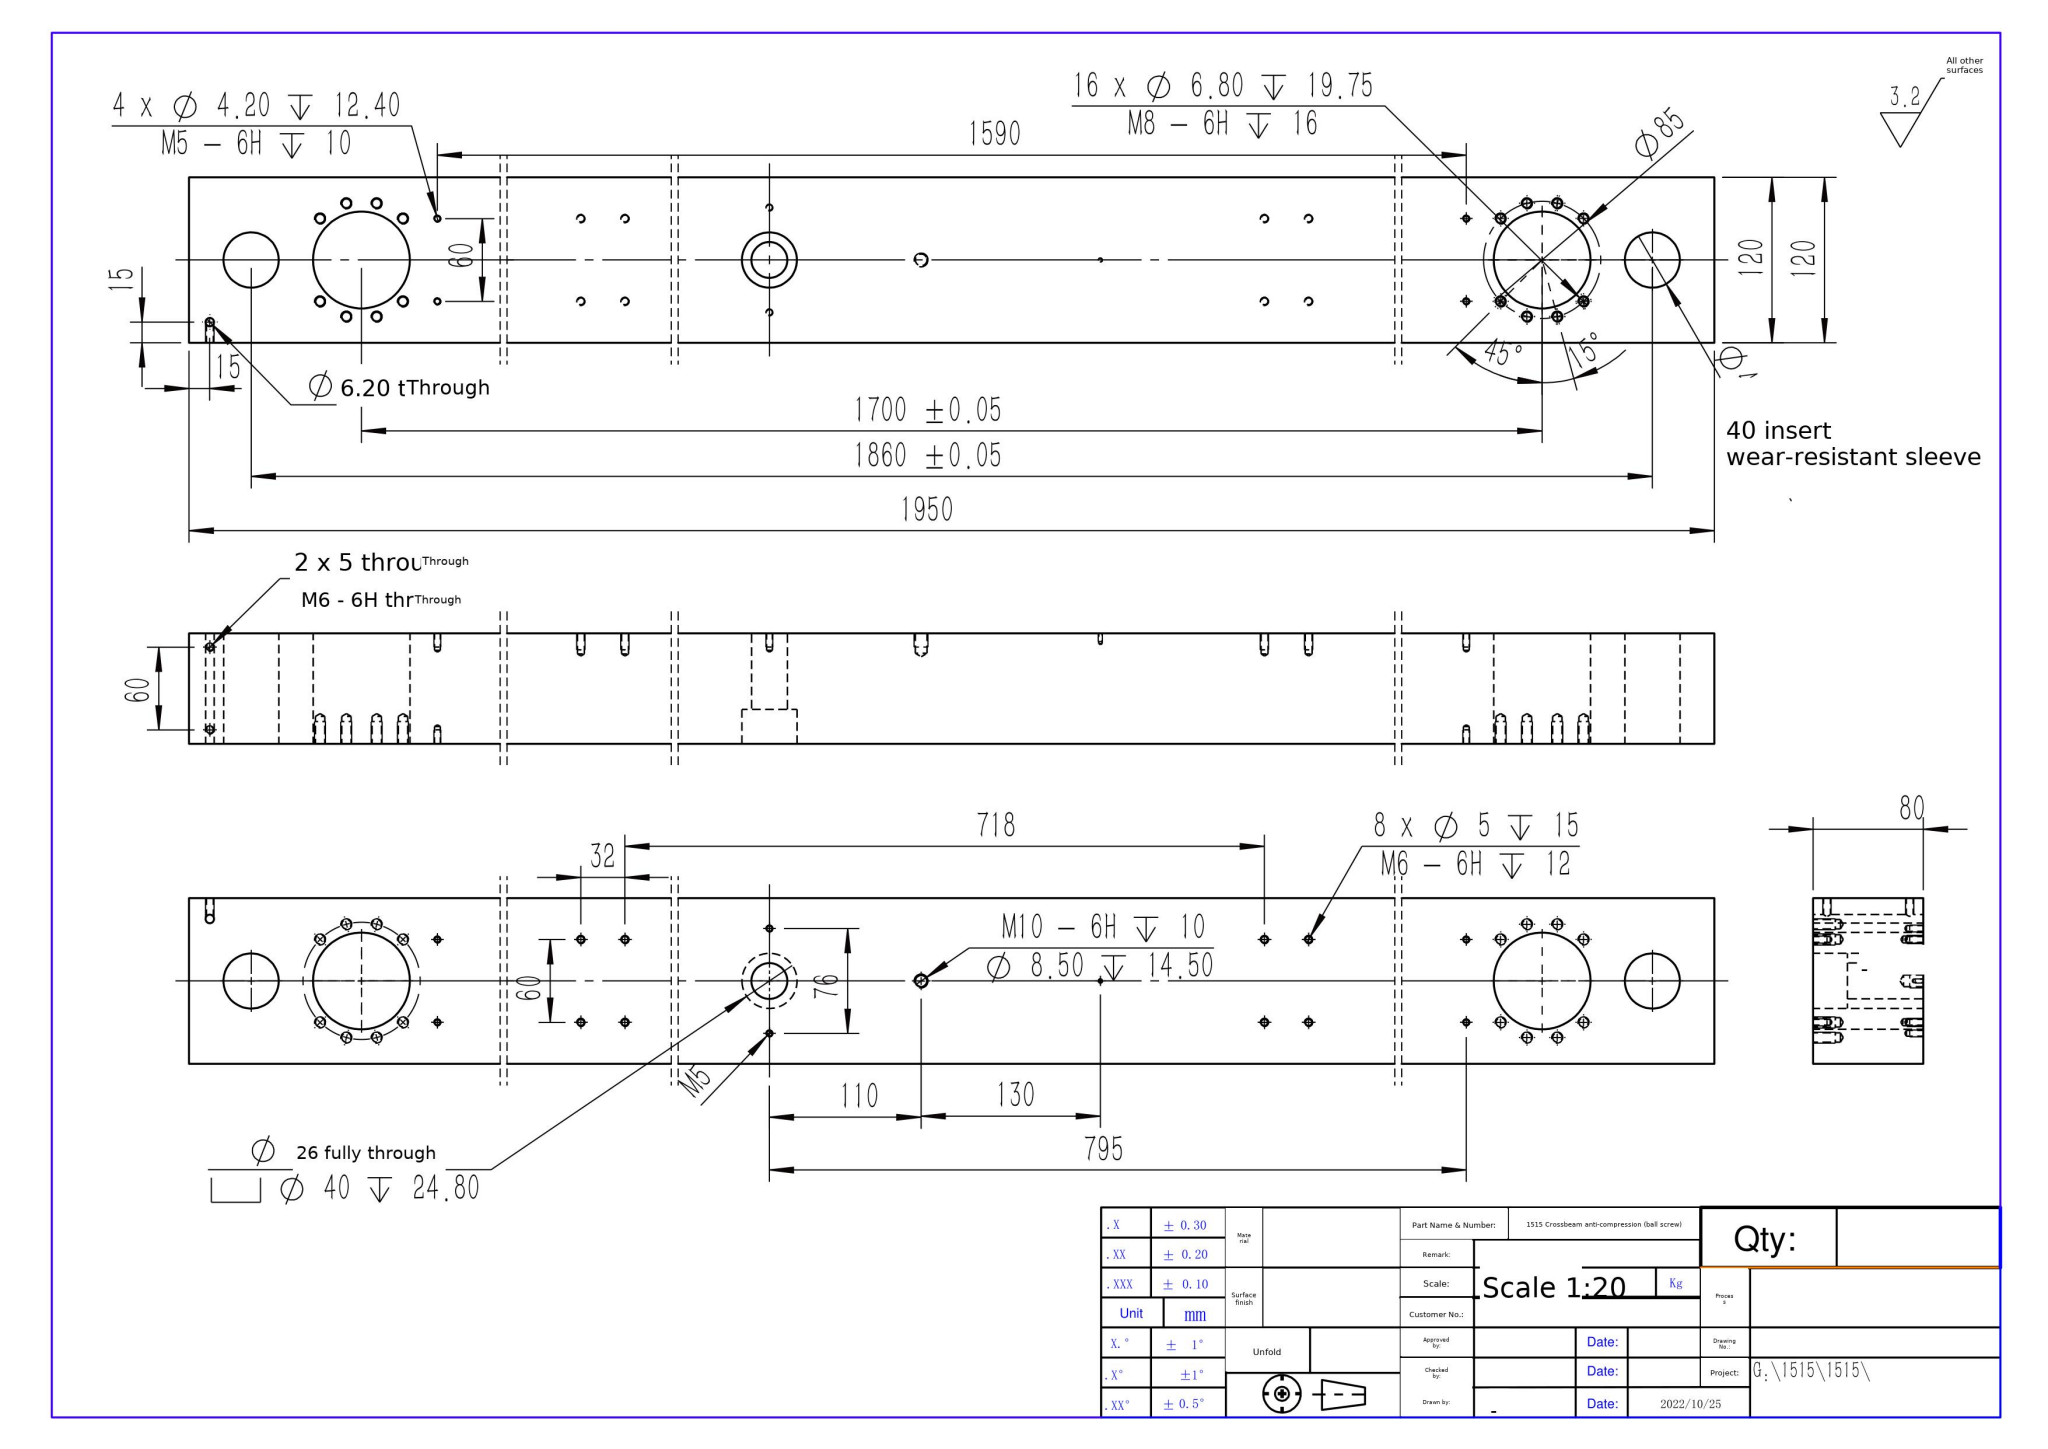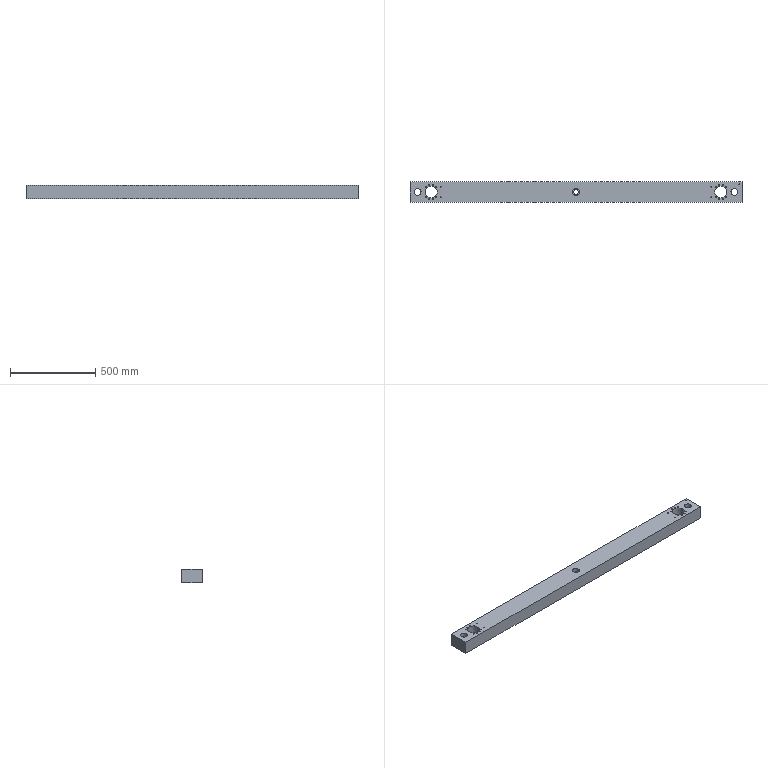Part | SolidWorks | mm | 1 solid | 169 faces | box 1950 x 120 x 80 mm | volume 17819305 mm3 | cylinder 90 | cone 72 | plane 7 | commonest cylinder face diameters 6.8 x32 4.2 x20 5 x20 40 x6 70.2 x4 26 x2 8.5 x2 6.2 x2
build123d program:
from build123d import *

# Parameters (mm, degrees)
SKETCH1_W                                        = 1950
SKETCH1_H                                        = 120
SKETCH1_R                                        = 20
SKETCH1_R_2                                      = 35.1
EXTRUDE1_DEPTH                                   = 40
M6_TAPPED_HOLE1_D                                = 5
M6_TAPPED_HOLE1_DEPTH                            = 15
M6_TAPPED_HOLE1_TIP                              = 1.502
M8_TAPPED_HOLE1_AT_2_COUNT                       = 2
M8_TAPPED_HOLE1_AT_2_PITCH                       = 60.104
M8_TAPPED_HOLE1_AT_3_COUNT                       = 2
M8_TAPPED_HOLE1_AT_3_PITCH                       = 85
M8_TAPPED_HOLE1_AT_4_COUNT                       = 2
M8_TAPPED_HOLE1_AT_4_PITCH                       = 82.104
M8_TAPPED_HOLE1_AT_5_COUNT                       = 2
M8_TAPPED_HOLE1_AT_5_PITCH                       = 73.612
M8_TAPPED_HOLE1_AT_6_COUNT                       = 2
M8_TAPPED_HOLE1_AT_6_PITCH                       = 22
M8_TAPPED_HOLE1_AT_7_COUNT                       = 2
M8_TAPPED_HOLE1_AT_7_PITCH                       = 42.5
M8_TAPPED_HOLE1_AT_8_COUNT                       = 2
M8_TAPPED_HOLE1_AT_8_PITCH                       = 60.104
M3_TAPPED_HOLE1_D                                = 2.5
M3_TAPPED_HOLE1_DEPTH                            = 7.5
M3_TAPPED_HOLE1_TIP                              = 0.7511
SKETCH31_R                                       = 3.1
CUT_EXTRUDE8_DEPTH                               = 981.115
M6_TAPPED_HOLE2_REACH                            = 985.171
M6_TAPPED_HOLE2_BORE_R                           = 2.5
M5_TAPPED_HOLE1_D                                = 4.2
M5_TAPPED_HOLE1_DEPTH                            = 12.4
M5_TAPPED_HOLE1_TIP                              = 1.262
M5_TAPPED_HOLE2_D                                = 4.2
M5_TAPPED_HOLE2_DEPTH                            = 12.4
M5_TAPPED_HOLE2_TIP                              = 1.262
M10_TAPPED_HOLE1_D                               = 8.5
M10_TAPPED_HOLE1_DEPTH                           = 14.5
M10_TAPPED_HOLE1_TIP                             = 2.554
M24_HEX_SOCKET_HEAD_CAP_SCREW_CBORE2_D           = 26
M24_HEX_SOCKET_HEAD_CAP_SCREW_CBORE2_CBORE_D     = 40
M24_HEX_SOCKET_HEAD_CAP_SCREW_CBORE2_CBORE_DEPTH = 24.8
M5_TAPPED_HOLE3_D                                = 4.2
M5_TAPPED_HOLE3_DEPTH                            = 12.4
M5_TAPPED_HOLE3_TIP                              = 1.262


with BuildPart() as part:
    # Sketch1 → Extrude1 (new, symmetric)
    with BuildSketch(Plane.XY):
        Rectangle(SKETCH1_W, SKETCH1_H)
        with Locations((-930, 0)):
            Circle(SKETCH1_R, mode=Mode.SUBTRACT)
        with Locations((-850, 0)):
            Circle(SKETCH1_R_2, mode=Mode.SUBTRACT)
        with Locations(Location((850, 0, 0), (0, 0, 180))):
            Circle(SKETCH1_R_2, mode=Mode.SUBTRACT)
        with Locations(Location((930, 0, 0), (0, 0, 180))):
            Circle(SKETCH1_R, mode=Mode.SUBTRACT)
    extrude(amount=EXTRUDE1_DEPTH, both=True)

    # M6 Tapped Hole1
    with Locations(Plane(origin=(0, 0, -40), x_dir=(-1, 0, 0), z_dir=(0, 0, -1))):
        with Locations((-391, -30), (-359, -30), (-391, 30), (-359, 30), (359, 30), (391, 30), (359, -30), (391, -30)):
            Hole(M6_TAPPED_HOLE1_D / 2, depth=M6_TAPPED_HOLE1_DEPTH)
            with Locations((0, 0, -(M6_TAPPED_HOLE1_DEPTH + M6_TAPPED_HOLE1_TIP / 2))):  # 118° drill point
                Cone(0, M6_TAPPED_HOLE1_D / 2, M6_TAPPED_HOLE1_TIP, mode=Mode.SUBTRACT)

    # Sketch14 → M8 Tapped Hole1 (revolve, cut)
    with BuildSketch(Plane(origin=(880.052, -30.052, 40), x_dir=(0, -1, 0), z_dir=(1, 0, 0))):
        Polygon((0, 0), (0, 21.793), (3.4, 19.75), (3.4, 0), align=None)
    m8_tapped_hole1 = revolve(axis=Axis((880.052, -30.052, 46.35), (0, 0, -1)), mode=Mode.SUBTRACT)

    # M8 Tapped Hole1 at 2: M8 Tapped Hole1 ×2
    with Locations(*[(0, i * M8_TAPPED_HOLE1_AT_2_PITCH, 0) for i in range(1, M8_TAPPED_HOLE1_AT_2_COUNT)]):
        add(m8_tapped_hole1, mode=Mode.SUBTRACT)

    # M8 Tapped Hole1 at 3: M8 Tapped Hole1 ×2
    with Locations(*[Vector(-0.7071, 0.7071, 0) * (i * M8_TAPPED_HOLE1_AT_3_PITCH) for i in range(1, M8_TAPPED_HOLE1_AT_3_COUNT)]):
        add(m8_tapped_hole1, mode=Mode.SUBTRACT)

    # M8 Tapped Hole1 at 4: M8 Tapped Hole1 ×2
    with Locations(*[Vector(-0.5, 0.866, 0) * (i * M8_TAPPED_HOLE1_AT_4_PITCH) for i in range(1, M8_TAPPED_HOLE1_AT_4_COUNT)]):
        add(m8_tapped_hole1, mode=Mode.SUBTRACT)

    # M8 Tapped Hole1 at 5: M8 Tapped Hole1 ×2
    with Locations(*[Vector(-0.2588, 0.9659, 0) * (i * M8_TAPPED_HOLE1_AT_5_PITCH) for i in range(1, M8_TAPPED_HOLE1_AT_5_COUNT)]):
        add(m8_tapped_hole1, mode=Mode.SUBTRACT)

    # M8 Tapped Hole1 at 6: M8 Tapped Hole1 ×2
    with Locations(*[Vector(-0.866, -0.5, 0) * (i * M8_TAPPED_HOLE1_AT_6_PITCH) for i in range(1, M8_TAPPED_HOLE1_AT_6_COUNT)]):
        add(m8_tapped_hole1, mode=Mode.SUBTRACT)

    # M8 Tapped Hole1 at 7: M8 Tapped Hole1 ×2
    with Locations(*[Vector(-0.9659, -0.2588, 0) * (i * M8_TAPPED_HOLE1_AT_7_PITCH) for i in range(1, M8_TAPPED_HOLE1_AT_7_COUNT)]):
        add(m8_tapped_hole1, mode=Mode.SUBTRACT)

    # M8 Tapped Hole1 at 8: M8 Tapped Hole1 ×2
    with Locations(*[(-i * M8_TAPPED_HOLE1_AT_8_PITCH, 0, 0) for i in range(1, M8_TAPPED_HOLE1_AT_8_COUNT)]):
        add(m8_tapped_hole1, mode=Mode.SUBTRACT)

    # Mirror3: M8 Tapped Hole1 across plane
    add(m8_tapped_hole1.mirror(Plane(origin=(0, 0, 0), x_dir=(0, 0, 1), z_dir=(1, 0, 0))), mode=Mode.SUBTRACT)

    # Mirror3 copy 1 sketch → Mirror3 copy 1 (revolve, cut)
    with BuildSketch(Plane(origin=(-880.052, 30.052, 40), x_dir=(0, -1, 0), z_dir=(-1, 0, 0))):
        Polygon((0, 0), (0, -21.793), (3.4, -19.75), (3.4, 0), align=None)
    revolve(axis=Axis((-880.052, 30.052, 46.35), (0, 0, 1)), mode=Mode.SUBTRACT)

    # Mirror3 copy 2 sketch → Mirror3 copy 2 (revolve, cut)
    with BuildSketch(Plane(origin=(-819.948, 30.052, 40), x_dir=(0, -1, 0), z_dir=(-1, 0, 0))):
        Polygon((0, 0), (0, -21.793), (3.4, -19.75), (3.4, 0), align=None)
    revolve(axis=Axis((-819.948, 30.052, 46.35), (0, 0, 1)), mode=Mode.SUBTRACT)

    # Mirror3 copy 3 sketch → Mirror3 copy 3 (revolve, cut)
    with BuildSketch(Plane(origin=(-839, 41.052, 40), x_dir=(0, -1, 0), z_dir=(-1, 0, 0))):
        Polygon((0, 0), (0, -21.793), (3.4, -19.75), (3.4, 0), align=None)
    revolve(axis=Axis((-839, 41.052, 46.35), (0, 0, 1)), mode=Mode.SUBTRACT)

    # Mirror3 copy 4 sketch → Mirror3 copy 4 (revolve, cut)
    with BuildSketch(Plane(origin=(-861, 41.052, 40), x_dir=(0, -1, 0), z_dir=(-1, 0, 0))):
        Polygon((0, 0), (0, -21.793), (3.4, -19.75), (3.4, 0), align=None)
    revolve(axis=Axis((-861, 41.052, 46.35), (0, 0, 1)), mode=Mode.SUBTRACT)

    # Mirror3 copy 5 sketch → Mirror3 copy 5 (revolve, cut)
    with BuildSketch(Plane(origin=(-861, -41.052, 40), x_dir=(0, -1, 0), z_dir=(-1, 0, 0))):
        Polygon((0, 0), (0, -21.793), (3.4, -19.75), (3.4, 0), align=None)
    revolve(axis=Axis((-861, -41.052, 46.35), (0, 0, 1)), mode=Mode.SUBTRACT)

    # Mirror3 copy 6 sketch → Mirror3 copy 6 (revolve, cut)
    with BuildSketch(Plane(origin=(-839, -41.052, 40), x_dir=(0, -1, 0), z_dir=(-1, 0, 0))):
        Polygon((0, 0), (0, -21.793), (3.4, -19.75), (3.4, 0), align=None)
    revolve(axis=Axis((-839, -41.052, 46.35), (0, 0, 1)), mode=Mode.SUBTRACT)

    # Mirror3 copy 7 sketch → Mirror3 copy 7 (revolve, cut)
    with BuildSketch(Plane(origin=(-819.948, -30.052, 40), x_dir=(0, -1, 0), z_dir=(-1, 0, 0))):
        Polygon((0, 0), (0, -21.793), (3.4, -19.75), (3.4, 0), align=None)
    revolve(axis=Axis((-819.948, -30.052, 46.35), (0, 0, 1)), mode=Mode.SUBTRACT)

    # M3 Tapped Hole1
    with Locations(Plane(origin=(0, 0, -40), x_dir=(-1, 0, 0), z_dir=(0, 0, -1))):
        with Locations((240, 0), (110, 0)):
            Hole(M3_TAPPED_HOLE1_D / 2, depth=M3_TAPPED_HOLE1_DEPTH)
            with Locations((0, 0, -(M3_TAPPED_HOLE1_DEPTH + M3_TAPPED_HOLE1_TIP / 2))):  # 118° drill point
                Cone(0, M3_TAPPED_HOLE1_D / 2, M3_TAPPED_HOLE1_TIP, mode=Mode.SUBTRACT)

    # Sketch31 → Cut-Extrude8 (cut, through all)
    with BuildSketch(Plane.XY.offset(40)):
        with Locations((960, 45)):
            Circle(SKETCH31_R)
    extrude(amount=-CUT_EXTRUDE8_DEPTH, mode=Mode.SUBTRACT)

    # M6 Tapped Hole2 bore → M6 Tapped Hole2 (cut, up to next)
    with BuildSketch(Plane(origin=(0, 60, 0), x_dir=(-1, 0, 0), z_dir=(0, 1, 0)), mode=Mode.PRIVATE) as m6_tapped_hole2_sk1:
        with Locations((-960, 30)):
            Circle(M6_TAPPED_HOLE2_BORE_R)
    m6_tapped_hole2_tool1 = extrude(m6_tapped_hole2_sk1.sketch, amount=-M6_TAPPED_HOLE2_REACH, mode=Mode.PRIVATE) & part.part
    # M6 Tapped Hole2 bore → M6 Tapped Hole2 (cut, up to next)
    with BuildSketch(Plane(origin=(0, 60, 0), x_dir=(-1, 0, 0), z_dir=(0, 1, 0)), mode=Mode.PRIVATE) as m6_tapped_hole2_sk2:
        with Locations((-960, -30)):
            Circle(M6_TAPPED_HOLE2_BORE_R)
    m6_tapped_hole2_tool2 = extrude(m6_tapped_hole2_sk2.sketch, amount=-M6_TAPPED_HOLE2_REACH, mode=Mode.PRIVATE) & part.part
    add(m6_tapped_hole2_tool1.solids().sort_by_distance((960, 60, 30))[0], mode=Mode.SUBTRACT)
    add(m6_tapped_hole2_tool2.solids().sort_by_distance((960, 60, -30))[0], mode=Mode.SUBTRACT)

    # M5 Tapped Hole1
    with Locations(Plane(origin=(0, 0, -40), x_dir=(-1, 0, 0), z_dir=(0, 0, -1))):
        with Locations((-795, 30), (-795, -30), (795, -30), (795, 30)):
            Hole(M5_TAPPED_HOLE1_D / 2, depth=M5_TAPPED_HOLE1_DEPTH)
            with Locations((0, 0, -(M5_TAPPED_HOLE1_DEPTH + M5_TAPPED_HOLE1_TIP / 2))):  # 118° drill point
                Cone(0, M5_TAPPED_HOLE1_D / 2, M5_TAPPED_HOLE1_TIP, mode=Mode.SUBTRACT)

    # M5 Tapped Hole2
    with Locations(Plane.XY.offset(40)):
        with Locations((795, 30), (795, -30), (-795, 30), (-795, -30)):
            Hole(M5_TAPPED_HOLE2_D / 2, depth=M5_TAPPED_HOLE2_DEPTH)
            with Locations((0, 0, -(M5_TAPPED_HOLE2_DEPTH + M5_TAPPED_HOLE2_TIP / 2))):  # 118° drill point
                Cone(0, M5_TAPPED_HOLE2_D / 2, M5_TAPPED_HOLE2_TIP, mode=Mode.SUBTRACT)

    # M10 Tapped Hole1
    with Locations(Plane(origin=(0, 0, -40), x_dir=(-1, 0, 0), z_dir=(0, 0, -1))):
        with Locations((110, 0)):
            Hole(M10_TAPPED_HOLE1_D / 2, depth=M10_TAPPED_HOLE1_DEPTH)
            with Locations((0, 0, -(M10_TAPPED_HOLE1_DEPTH + M10_TAPPED_HOLE1_TIP / 2))):  # 118° drill point
                Cone(0, M10_TAPPED_HOLE1_D / 2, M10_TAPPED_HOLE1_TIP, mode=Mode.SUBTRACT)

    # M24 Hex Socket Head Cap Screw CBORE2 (through all)
    with Locations(Plane.XY.offset(40)):
        with Locations((0, 0)):
            CounterBoreHole(M24_HEX_SOCKET_HEAD_CAP_SCREW_CBORE2_D / 2, M24_HEX_SOCKET_HEAD_CAP_SCREW_CBORE2_CBORE_D / 2, M24_HEX_SOCKET_HEAD_CAP_SCREW_CBORE2_CBORE_DEPTH)

    # M5 Tapped Hole3
    with Locations(Plane(origin=(0, 0, -40), x_dir=(-1, 0, 0), z_dir=(0, 0, -1))):
        with Locations((0, 38), (0, -38)):
            Hole(M5_TAPPED_HOLE3_D / 2, depth=M5_TAPPED_HOLE3_DEPTH)
            with Locations((0, 0, -(M5_TAPPED_HOLE3_DEPTH + M5_TAPPED_HOLE3_TIP / 2))):  # 118° drill point
                Cone(0, M5_TAPPED_HOLE3_D / 2, M5_TAPPED_HOLE3_TIP, mode=Mode.SUBTRACT)


solid = part.part